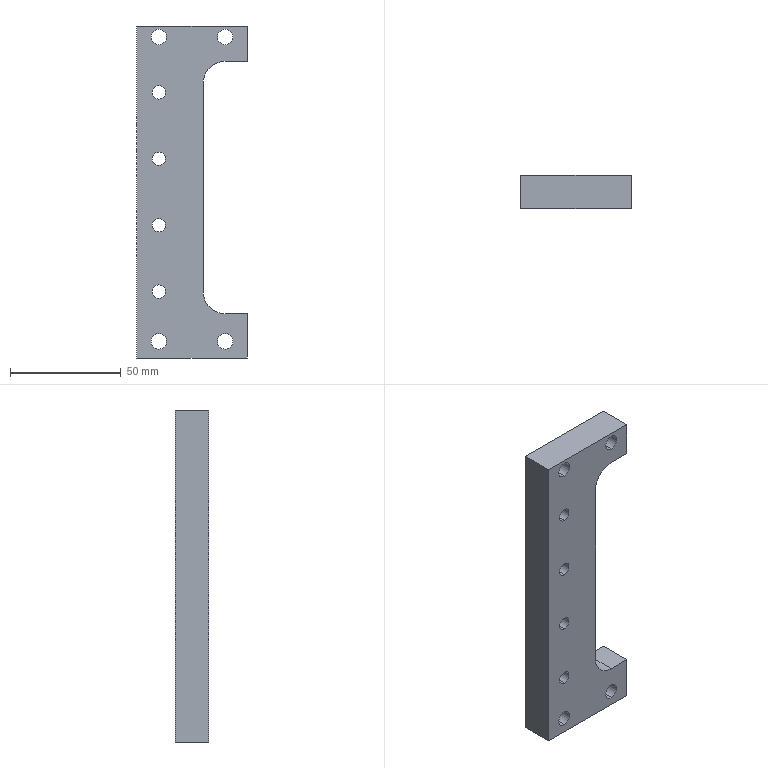Component | SolidWorks | JL001-05-05-001-1 | 1 solid | 28 faces | box 50 x 15 x 150 mm | volume 74938 mm3 | cylinder 18 | plane 10 | commonest cylinder face diameters 7 x8 6 x8 20 x2
build123d program:
from build123d import *

# Parameters (mm, degrees)
SKETCH1_W                    = 50
SKETCH1_H                    = 150
BOSS_EXTRUDE1_DEPTH          = 15
M6_TAPPED_HOLE1_D            = 6
F_7_0_7_DIAMETER_HOLE1_D     = 7
F_7_0_7_DIAMETER_HOLE1_DEPTH = 15
F_7_0_7_DIAMETER_HOLE1_TIP   = 2.103
SKETCH6_W                    = 20
SKETCH6_H                    = 114
CUT_EXTRUDE1_DEPTH           = 81.467
FILLET1_R                    = 10


with BuildPart() as part:
    # Sketch1 → Boss-Extrude1 (new body)
    with BuildSketch(Plane(origin=(0, 0, 0), x_dir=(1, 0, 0), z_dir=(0, 1, 0))):
        Rectangle(SKETCH1_W, SKETCH1_H)
    extrude(amount=BOSS_EXTRUDE1_DEPTH)

    # M6 Tapped Hole1 (through all)
    with Locations(Plane(origin=(0, 15, 0), x_dir=(1, 0, 0), z_dir=(0, 1, 0))):
        with Locations((-15, -15), (-15, -45), (-15, 15), (-15, 45)):
            Hole(M6_TAPPED_HOLE1_D / 2)

    # 7.0 _7_ Diameter Hole1
    with Locations(Plane(origin=(0, 15, 0), x_dir=(1, 0, 0), z_dir=(0, 1, 0))):
        with Locations((-15, -70), (15, -70), (-15, 67.5), (15, 67.5)):
            Hole(F_7_0_7_DIAMETER_HOLE1_D / 2, depth=F_7_0_7_DIAMETER_HOLE1_DEPTH)
            with Locations((0, 0, -(F_7_0_7_DIAMETER_HOLE1_DEPTH + F_7_0_7_DIAMETER_HOLE1_TIP / 2))):  # 118° drill point
                Cone(0, F_7_0_7_DIAMETER_HOLE1_D / 2, F_7_0_7_DIAMETER_HOLE1_TIP, mode=Mode.SUBTRACT)

    # Sketch6 → Cut-Extrude1 (cut, through all)
    with BuildSketch(Plane(origin=(0, 15, 0), x_dir=(1, 0, 0), z_dir=(0, 1, 0))):
        with Locations((15, -2)):
            Rectangle(SKETCH6_W, SKETCH6_H)
    extrude(amount=-CUT_EXTRUDE1_DEPTH, mode=Mode.SUBTRACT)

    # Fillet1
    fillet1_edges = [part.edges().sort_by_distance(p)[0] for p in [
        (5, 7.5, 59),
        (5, 7.5, -55),
    ]]
    fillet(fillet1_edges, radius=FILLET1_R)


solid = part.part

# Placed as in the assembly
solid = solid.moved(Location((0, -52.5, 67.5), (0, 0, 0)))
STEP:
#1=COLOUR_RGB('',0.7922,0.8196,0.9333);
#2=FILL_AREA_STYLE_COLOUR('',#1);
#3=FILL_AREA_STYLE('',(#2));
#4=SURFACE_STYLE_FILL_AREA(#3);
#5=SURFACE_SIDE_STYLE('',(#4));
#6=SURFACE_STYLE_USAGE(.BOTH.,#5);
#7=PRESENTATION_STYLE_ASSIGNMENT((#6));
#8=CARTESIAN_POINT('',(-0.5906,-2.067,5.276));
#9=VERTEX_POINT('',#8);
#10=CARTESIAN_POINT('',(-0.5906,-2.067,5.551));
#11=VERTEX_POINT('',#10);
#12=CARTESIAN_POINT('',(-0.5906,-2.067,5.413));
#13=DIRECTION('',(0.,1.,0.));
#14=DIRECTION('',(0.,0.,1.));
#15=AXIS2_PLACEMENT_3D('',#12,#13,#14);
#16=CIRCLE('',#15,0.1378);
#17=EDGE_CURVE('',#9,#11,#16,.T.);
#18=ORIENTED_EDGE('',*,*,#17,.F.);
#19=CARTESIAN_POINT('',(-0.5906,-1.476,5.276));
#20=VERTEX_POINT('',#19);
#21=CARTESIAN_POINT('',(-0.5906,-1.476,5.276));
#22=DIRECTION('',(0.,1.,0.));
#23=VECTOR('',#22,39.37);
#24=LINE('',#21,#23);
#25=EDGE_CURVE('',#9,#20,#24,.T.);
#26=ORIENTED_EDGE('',*,*,#25,.T.);
#27=CARTESIAN_POINT('',(-0.5906,-1.476,5.551));
#28=VERTEX_POINT('',#27);
#29=CARTESIAN_POINT('',(-0.5906,-1.476,5.413));
#30=DIRECTION('',(0.,1.,0.));
#31=DIRECTION('',(0.,0.,1.));
#32=AXIS2_PLACEMENT_3D('',#29,#30,#31);
#33=CIRCLE('',#32,0.1378);
#34=EDGE_CURVE('',#20,#28,#33,.T.);
#35=ORIENTED_EDGE('',*,*,#34,.T.);
#36=CARTESIAN_POINT('',(-0.5906,-1.476,5.551));
#37=DIRECTION('',(0.,1.,0.));
#38=VECTOR('',#37,39.37);
#39=LINE('',#36,#38);
#40=EDGE_CURVE('',#11,#28,#39,.T.);
#41=ORIENTED_EDGE('',*,*,#40,.F.);
#42=EDGE_LOOP('',(#18,#26,#35,#41));
#43=FACE_OUTER_BOUND('',#42,.T.);
#44=CARTESIAN_POINT('',(-0.5906,-1.476,5.413));
#45=DIRECTION('',(0.,1.,0.));
#46=DIRECTION('',(0.,0.,1.));
#47=AXIS2_PLACEMENT_3D('',#44,#45,#46);
#48=CYLINDRICAL_SURFACE('',#47,0.1378);
#49=ADVANCED_FACE('',(#43),#48,.F.);
#50=CARTESIAN_POINT('',(0.5906,-2.067,5.276));
#51=VERTEX_POINT('',#50);
#52=CARTESIAN_POINT('',(0.5906,-2.067,5.551));
#53=VERTEX_POINT('',#52);
#54=CARTESIAN_POINT('',(0.5906,-2.067,5.413));
#55=DIRECTION('',(0.,1.,0.));
#56=DIRECTION('',(0.,0.,1.));
#57=AXIS2_PLACEMENT_3D('',#54,#55,#56);
#58=CIRCLE('',#57,0.1378);
#59=EDGE_CURVE('',#51,#53,#58,.T.);
#60=ORIENTED_EDGE('',*,*,#59,.F.);
#61=CARTESIAN_POINT('',(0.5906,-1.476,5.276));
#62=VERTEX_POINT('',#61);
#63=CARTESIAN_POINT('',(0.5906,-1.476,5.276));
#64=DIRECTION('',(0.,1.,0.));
#65=VECTOR('',#64,39.37);
#66=LINE('',#63,#65);
#67=EDGE_CURVE('',#51,#62,#66,.T.);
#68=ORIENTED_EDGE('',*,*,#67,.T.);
#69=CARTESIAN_POINT('',(0.5906,-1.476,5.551));
#70=VERTEX_POINT('',#69);
#71=CARTESIAN_POINT('',(0.5906,-1.476,5.413));
#72=DIRECTION('',(0.,1.,0.));
#73=DIRECTION('',(0.,0.,1.));
#74=AXIS2_PLACEMENT_3D('',#71,#72,#73);
#75=CIRCLE('',#74,0.1378);
#76=EDGE_CURVE('',#62,#70,#75,.T.);
#77=ORIENTED_EDGE('',*,*,#76,.T.);
#78=CARTESIAN_POINT('',(0.5906,-1.476,5.551));
#79=DIRECTION('',(0.,1.,0.));
#80=VECTOR('',#79,39.37);
#81=LINE('',#78,#80);
#82=EDGE_CURVE('',#53,#70,#81,.T.);
#83=ORIENTED_EDGE('',*,*,#82,.F.);
#84=EDGE_LOOP('',(#60,#68,#77,#83));
#85=FACE_OUTER_BOUND('',#84,.T.);
#86=CARTESIAN_POINT('',(0.5906,-1.476,5.413));
#87=DIRECTION('',(0.,1.,0.));
#88=DIRECTION('',(0.,0.,1.));
#89=AXIS2_PLACEMENT_3D('',#86,#87,#88);
#90=CYLINDRICAL_SURFACE('',#89,0.1378);
#91=ADVANCED_FACE('',(#85),#90,.F.);
#92=CARTESIAN_POINT('',(-0.5906,-2.067,-0.1378));
#93=VERTEX_POINT('',#92);
#94=CARTESIAN_POINT('',(-0.5906,-2.067,0.1378));
#95=VERTEX_POINT('',#94);
#96=CARTESIAN_POINT('',(-0.5906,-2.067,0.));
#97=DIRECTION('',(0.,1.,0.));
#98=DIRECTION('',(0.,0.,1.));
#99=AXIS2_PLACEMENT_3D('',#96,#97,#98);
#100=CIRCLE('',#99,0.1378);
#101=EDGE_CURVE('',#93,#95,#100,.T.);
#102=ORIENTED_EDGE('',*,*,#101,.F.);
#103=CARTESIAN_POINT('',(-0.5906,-1.476,-0.1378));
#104=VERTEX_POINT('',#103);
#105=CARTESIAN_POINT('',(-0.5906,-1.476,-0.1378));
#106=DIRECTION('',(0.,1.,0.));
#107=VECTOR('',#106,39.37);
#108=LINE('',#105,#107);
#109=EDGE_CURVE('',#93,#104,#108,.T.);
#110=ORIENTED_EDGE('',*,*,#109,.T.);
#111=CARTESIAN_POINT('',(-0.5906,-1.476,0.1378));
#112=VERTEX_POINT('',#111);
#113=CARTESIAN_POINT('',(-0.5906,-1.476,0.));
#114=DIRECTION('',(0.,1.,0.));
#115=DIRECTION('',(0.,0.,1.));
#116=AXIS2_PLACEMENT_3D('',#113,#114,#115);
#117=CIRCLE('',#116,0.1378);
#118=EDGE_CURVE('',#104,#112,#117,.T.);
#119=ORIENTED_EDGE('',*,*,#118,.T.);
#120=CARTESIAN_POINT('',(-0.5906,-1.476,0.1378));
#121=DIRECTION('',(0.,1.,0.));
#122=VECTOR('',#121,39.37);
#123=LINE('',#120,#122);
#124=EDGE_CURVE('',#95,#112,#123,.T.);
#125=ORIENTED_EDGE('',*,*,#124,.F.);
#126=EDGE_LOOP('',(#102,#110,#119,#125));
#127=FACE_OUTER_BOUND('',#126,.T.);
#128=CARTESIAN_POINT('',(-0.5906,-1.476,0.));
#129=DIRECTION('',(0.,1.,0.));
#130=DIRECTION('',(0.,0.,1.));
#131=AXIS2_PLACEMENT_3D('',#128,#129,#130);
#132=CYLINDRICAL_SURFACE('',#131,0.1378);
#133=ADVANCED_FACE('',(#127),#132,.F.);
#134=CARTESIAN_POINT('',(0.5906,-2.067,-0.1378));
#135=VERTEX_POINT('',#134);
#136=CARTESIAN_POINT('',(0.5906,-2.067,0.1378));
#137=VERTEX_POINT('',#136);
#138=CARTESIAN_POINT('',(0.5906,-2.067,0.));
#139=DIRECTION('',(0.,1.,0.));
#140=DIRECTION('',(0.,0.,1.));
#141=AXIS2_PLACEMENT_3D('',#138,#139,#140);
#142=CIRCLE('',#141,0.1378);
#143=EDGE_CURVE('',#135,#137,#142,.T.);
#144=ORIENTED_EDGE('',*,*,#143,.F.);
#145=CARTESIAN_POINT('',(0.5906,-1.476,-0.1378));
#146=VERTEX_POINT('',#145);
#147=CARTESIAN_POINT('',(0.5906,-1.476,-0.1378));
#148=DIRECTION('',(0.,1.,0.));
#149=VECTOR('',#148,39.37);
#150=LINE('',#147,#149);
#151=EDGE_CURVE('',#135,#146,#150,.T.);
#152=ORIENTED_EDGE('',*,*,#151,.T.);
#153=CARTESIAN_POINT('',(0.5906,-1.476,0.1378));
#154=VERTEX_POINT('',#153);
#155=CARTESIAN_POINT('',(0.5906,-1.476,0.));
#156=DIRECTION('',(0.,1.,0.));
#157=DIRECTION('',(0.,0.,1.));
#158=AXIS2_PLACEMENT_3D('',#155,#156,#157);
#159=CIRCLE('',#158,0.1378);
#160=EDGE_CURVE('',#146,#154,#159,.T.);
#161=ORIENTED_EDGE('',*,*,#160,.T.);
#162=CARTESIAN_POINT('',(0.5906,-1.476,0.1378));
#163=DIRECTION('',(0.,1.,0.));
#164=VECTOR('',#163,39.37);
#165=LINE('',#162,#164);
#166=EDGE_CURVE('',#137,#154,#165,.T.);
#167=ORIENTED_EDGE('',*,*,#166,.F.);
#168=EDGE_LOOP('',(#144,#152,#161,#167));
#169=FACE_OUTER_BOUND('',#168,.T.);
#170=CARTESIAN_POINT('',(0.5906,-1.476,0.));
#171=DIRECTION('',(0.,1.,0.));
#172=DIRECTION('',(0.,0.,1.));
#173=AXIS2_PLACEMENT_3D('',#170,#171,#172);
#174=CYLINDRICAL_SURFACE('',#173,0.1378);
#175=ADVANCED_FACE('',(#169),#174,.F.);
#176=CARTESIAN_POINT('',(-0.5906,-2.067,3.13));
#177=VERTEX_POINT('',#176);
#178=CARTESIAN_POINT('',(-0.5906,-2.067,3.366));
#179=VERTEX_POINT('',#178);
#180=CARTESIAN_POINT('',(-0.5906,-2.067,3.248));
#181=DIRECTION('',(0.,1.,0.));
#182=DIRECTION('',(0.,0.,1.));
#183=AXIS2_PLACEMENT_3D('',#180,#181,#182);
#184=CIRCLE('',#183,0.1181);
#185=EDGE_CURVE('',#177,#179,#184,.T.);
#186=ORIENTED_EDGE('',*,*,#185,.F.);
#187=CARTESIAN_POINT('',(-0.5906,-1.476,3.13));
#188=VERTEX_POINT('',#187);
#189=CARTESIAN_POINT('',(-0.5906,-1.476,3.13));
#190=DIRECTION('',(0.,1.,0.));
#191=VECTOR('',#190,39.37);
#192=LINE('',#189,#191);
#193=EDGE_CURVE('',#177,#188,#192,.T.);
#194=ORIENTED_EDGE('',*,*,#193,.T.);
#195=CARTESIAN_POINT('',(-0.5906,-1.476,3.366));
#196=VERTEX_POINT('',#195);
#197=CARTESIAN_POINT('',(-0.5906,-1.476,3.248));
#198=DIRECTION('',(0.,1.,0.));
#199=DIRECTION('',(0.,0.,1.));
#200=AXIS2_PLACEMENT_3D('',#197,#198,#199);
#201=CIRCLE('',#200,0.1181);
#202=EDGE_CURVE('',#188,#196,#201,.T.);
#203=ORIENTED_EDGE('',*,*,#202,.T.);
#204=CARTESIAN_POINT('',(-0.5906,-1.476,3.366));
#205=DIRECTION('',(0.,1.,0.));
#206=VECTOR('',#205,39.37);
#207=LINE('',#204,#206);
#208=EDGE_CURVE('',#179,#196,#207,.T.);
#209=ORIENTED_EDGE('',*,*,#208,.F.);
#210=EDGE_LOOP('',(#186,#194,#203,#209));
#211=FACE_OUTER_BOUND('',#210,.T.);
#212=CARTESIAN_POINT('',(-0.5906,-1.476,3.248));
#213=DIRECTION('',(0.,1.,0.));
#214=DIRECTION('',(0.,0.,1.));
#215=AXIS2_PLACEMENT_3D('',#212,#213,#214);
#216=CYLINDRICAL_SURFACE('',#215,0.1181);
#217=ADVANCED_FACE('',(#211),#216,.F.);
#218=CARTESIAN_POINT('',(-0.5906,-2.067,4.311));
#219=VERTEX_POINT('',#218);
#220=CARTESIAN_POINT('',(-0.5906,-2.067,4.547));
#221=VERTEX_POINT('',#220);
#222=CARTESIAN_POINT('',(-0.5906,-2.067,4.429));
#223=DIRECTION('',(0.,1.,0.));
#224=DIRECTION('',(0.,0.,1.));
#225=AXIS2_PLACEMENT_3D('',#222,#223,#224);
#226=CIRCLE('',#225,0.1181);
#227=EDGE_CURVE('',#219,#221,#226,.T.);
#228=ORIENTED_EDGE('',*,*,#227,.F.);
#229=CARTESIAN_POINT('',(-0.5906,-1.476,4.311));
#230=VERTEX_POINT('',#229);
#231=CARTESIAN_POINT('',(-0.5906,-1.476,4.311));
#232=DIRECTION('',(0.,1.,0.));
#233=VECTOR('',#232,39.37);
#234=LINE('',#231,#233);
#235=EDGE_CURVE('',#219,#230,#234,.T.);
#236=ORIENTED_EDGE('',*,*,#235,.T.);
#237=CARTESIAN_POINT('',(-0.5906,-1.476,4.547));
#238=VERTEX_POINT('',#237);
#239=CARTESIAN_POINT('',(-0.5906,-1.476,4.429));
#240=DIRECTION('',(0.,1.,0.));
#241=DIRECTION('',(0.,0.,1.));
#242=AXIS2_PLACEMENT_3D('',#239,#240,#241);
#243=CIRCLE('',#242,0.1181);
#244=EDGE_CURVE('',#230,#238,#243,.T.);
#245=ORIENTED_EDGE('',*,*,#244,.T.);
#246=CARTESIAN_POINT('',(-0.5906,-1.476,4.547));
#247=DIRECTION('',(0.,1.,0.));
#248=VECTOR('',#247,39.37);
#249=LINE('',#246,#248);
#250=EDGE_CURVE('',#221,#238,#249,.T.);
#251=ORIENTED_EDGE('',*,*,#250,.F.);
#252=EDGE_LOOP('',(#228,#236,#245,#251));
#253=FACE_OUTER_BOUND('',#252,.T.);
#254=CARTESIAN_POINT('',(-0.5906,-1.476,4.429));
#255=DIRECTION('',(0.,1.,0.));
#256=DIRECTION('',(0.,0.,1.));
#257=AXIS2_PLACEMENT_3D('',#254,#255,#256);
#258=CYLINDRICAL_SURFACE('',#257,0.1181);
#259=ADVANCED_FACE('',(#253),#258,.F.);
#260=CARTESIAN_POINT('',(-0.5906,-2.067,1.949));
#261=VERTEX_POINT('',#260);
#262=CARTESIAN_POINT('',(-0.5906,-2.067,2.185));
#263=VERTEX_POINT('',#262);
#264=CARTESIAN_POINT('',(-0.5906,-2.067,2.067));
#265=DIRECTION('',(0.,1.,0.));
#266=DIRECTION('',(0.,0.,1.));
#267=AXIS2_PLACEMENT_3D('',#264,#265,#266);
#268=CIRCLE('',#267,0.1181);
#269=EDGE_CURVE('',#261,#263,#268,.T.);
#270=ORIENTED_EDGE('',*,*,#269,.F.);
#271=CARTESIAN_POINT('',(-0.5906,-1.476,1.949));
#272=VERTEX_POINT('',#271);
#273=CARTESIAN_POINT('',(-0.5906,-1.476,1.949));
#274=DIRECTION('',(0.,1.,0.));
#275=VECTOR('',#274,39.37);
#276=LINE('',#273,#275);
#277=EDGE_CURVE('',#261,#272,#276,.T.);
#278=ORIENTED_EDGE('',*,*,#277,.T.);
#279=CARTESIAN_POINT('',(-0.5906,-1.476,2.185));
#280=VERTEX_POINT('',#279);
#281=CARTESIAN_POINT('',(-0.5906,-1.476,2.067));
#282=DIRECTION('',(0.,1.,0.));
#283=DIRECTION('',(0.,0.,1.));
#284=AXIS2_PLACEMENT_3D('',#281,#282,#283);
#285=CIRCLE('',#284,0.1181);
#286=EDGE_CURVE('',#272,#280,#285,.T.);
#287=ORIENTED_EDGE('',*,*,#286,.T.);
#288=CARTESIAN_POINT('',(-0.5906,-1.476,2.185));
#289=DIRECTION('',(0.,1.,0.));
#290=VECTOR('',#289,39.37);
#291=LINE('',#288,#290);
#292=EDGE_CURVE('',#263,#280,#291,.T.);
#293=ORIENTED_EDGE('',*,*,#292,.F.);
#294=EDGE_LOOP('',(#270,#278,#287,#293));
#295=FACE_OUTER_BOUND('',#294,.T.);
#296=CARTESIAN_POINT('',(-0.5906,-1.476,2.067));
#297=DIRECTION('',(0.,1.,0.));
#298=DIRECTION('',(0.,0.,1.));
#299=AXIS2_PLACEMENT_3D('',#296,#297,#298);
#300=CYLINDRICAL_SURFACE('',#299,0.1181);
#301=ADVANCED_FACE('',(#295),#300,.F.);
#302=CARTESIAN_POINT('',(-0.5906,-2.067,0.7677));
#303=VERTEX_POINT('',#302);
#304=CARTESIAN_POINT('',(-0.5906,-2.067,1.004));
#305=VERTEX_POINT('',#304);
#306=CARTESIAN_POINT('',(-0.5906,-2.067,0.8858));
#307=DIRECTION('',(0.,1.,0.));
#308=DIRECTION('',(0.,0.,1.));
#309=AXIS2_PLACEMENT_3D('',#306,#307,#308);
#310=CIRCLE('',#309,0.1181);
#311=EDGE_CURVE('',#303,#305,#310,.T.);
#312=ORIENTED_EDGE('',*,*,#311,.F.);
#313=CARTESIAN_POINT('',(-0.5906,-1.476,0.7677));
#314=VERTEX_POINT('',#313);
#315=CARTESIAN_POINT('',(-0.5906,-1.476,0.7677));
#316=DIRECTION('',(0.,1.,0.));
#317=VECTOR('',#316,39.37);
#318=LINE('',#315,#317);
#319=EDGE_CURVE('',#303,#314,#318,.T.);
#320=ORIENTED_EDGE('',*,*,#319,.T.);
#321=CARTESIAN_POINT('',(-0.5906,-1.476,1.004));
#322=VERTEX_POINT('',#321);
#323=CARTESIAN_POINT('',(-0.5906,-1.476,0.8858));
#324=DIRECTION('',(0.,1.,0.));
#325=DIRECTION('',(0.,0.,1.));
#326=AXIS2_PLACEMENT_3D('',#323,#324,#325);
#327=CIRCLE('',#326,0.1181);
#328=EDGE_CURVE('',#314,#322,#327,.T.);
#329=ORIENTED_EDGE('',*,*,#328,.T.);
#330=CARTESIAN_POINT('',(-0.5906,-1.476,1.004));
#331=DIRECTION('',(0.,1.,0.));
#332=VECTOR('',#331,39.37);
#333=LINE('',#330,#332);
#334=EDGE_CURVE('',#305,#322,#333,.T.);
#335=ORIENTED_EDGE('',*,*,#334,.F.);
#336=EDGE_LOOP('',(#312,#320,#329,#335));
#337=FACE_OUTER_BOUND('',#336,.T.);
#338=CARTESIAN_POINT('',(-0.5906,-1.476,0.8858));
#339=DIRECTION('',(0.,1.,0.));
#340=DIRECTION('',(0.,0.,1.));
#341=AXIS2_PLACEMENT_3D('',#338,#339,#340);
#342=CYLINDRICAL_SURFACE('',#341,0.1181);
#343=ADVANCED_FACE('',(#337),#342,.F.);
#344=CARTESIAN_POINT('',(0.9843,-2.067,5.61));
#345=VERTEX_POINT('',#344);
#346=CARTESIAN_POINT('',(0.9843,-2.067,4.98));
#347=VERTEX_POINT('',#346);
#348=CARTESIAN_POINT('',(0.9843,-2.067,-0.2953));
#349=DIRECTION('',(-0.,0.,-1.));
#350=VECTOR('',#349,39.37);
#351=LINE('',#348,#350);
#352=EDGE_CURVE('',#345,#347,#351,.T.);
#353=ORIENTED_EDGE('',*,*,#352,.T.);
#354=CARTESIAN_POINT('',(0.9843,-1.476,4.98));
#355=VERTEX_POINT('',#354);
#356=CARTESIAN_POINT('',(0.9843,-2.067,4.98));
#357=DIRECTION('',(0.,1.,0.));
#358=VECTOR('',#357,39.37);
#359=LINE('',#356,#358);
#360=EDGE_CURVE('',#347,#355,#359,.T.);
#361=ORIENTED_EDGE('',*,*,#360,.T.);
#362=CARTESIAN_POINT('',(0.9843,-1.476,5.61));
#363=VERTEX_POINT('',#362);
#364=CARTESIAN_POINT('',(0.9843,-1.476,-0.2953));
#365=DIRECTION('',(-0.,0.,-1.));
#366=VECTOR('',#365,39.37);
#367=LINE('',#364,#366);
#368=EDGE_CURVE('',#363,#355,#367,.T.);
#369=ORIENTED_EDGE('',*,*,#368,.F.);
#370=CARTESIAN_POINT('',(0.9843,-1.476,5.61));
#371=DIRECTION('',(0.,-1.,0.));
#372=VECTOR('',#371,39.37);
#373=LINE('',#370,#372);
#374=EDGE_CURVE('',#363,#345,#373,.T.);
#375=ORIENTED_EDGE('',*,*,#374,.T.);
#376=EDGE_LOOP('',(#353,#361,#369,#375));
#377=FACE_OUTER_BOUND('',#376,.T.);
#378=CARTESIAN_POINT('',(0.9843,-1.476,-0.2953));
#379=DIRECTION('',(-1.,0.,0.));
#380=DIRECTION('',(0.,0.,1.));
#381=AXIS2_PLACEMENT_3D('',#378,#379,#380);
#382=PLANE('',#381);
#383=ADVANCED_FACE('',(#377),#382,.F.);
#384=CARTESIAN_POINT('',(0.9843,-1.476,0.4921));
#385=VERTEX_POINT('',#384);
#386=CARTESIAN_POINT('',(0.9843,-1.476,-0.2953));
#387=VERTEX_POINT('',#386);
#388=CARTESIAN_POINT('',(0.9843,-1.476,-0.2953));
#389=DIRECTION('',(-0.,0.,-1.));
#390=VECTOR('',#389,39.37);
#391=LINE('',#388,#390);
#392=EDGE_CURVE('',#385,#387,#391,.T.);
#393=ORIENTED_EDGE('',*,*,#392,.F.);
#394=CARTESIAN_POINT('',(0.9843,-2.067,0.4921));
#395=VERTEX_POINT('',#394);
#396=CARTESIAN_POINT('',(0.9843,-2.067,0.4921));
#397=DIRECTION('',(0.,1.,0.));
#398=VECTOR('',#397,39.37);
#399=LINE('',#396,#398);
#400=EDGE_CURVE('',#395,#385,#399,.T.);
#401=ORIENTED_EDGE('',*,*,#400,.F.);
#402=CARTESIAN_POINT('',(0.9843,-2.067,-0.2953));
#403=VERTEX_POINT('',#402);
#404=CARTESIAN_POINT('',(0.9843,-2.067,-0.2953));
#405=DIRECTION('',(-0.,0.,-1.));
#406=VECTOR('',#405,39.37);
#407=LINE('',#404,#406);
#408=EDGE_CURVE('',#395,#403,#407,.T.);
#409=ORIENTED_EDGE('',*,*,#408,.T.);
#410=CARTESIAN_POINT('',(0.9843,-1.476,-0.2953));
#411=DIRECTION('',(0.,-1.,0.));
#412=VECTOR('',#411,39.37);
#413=LINE('',#410,#412);
#414=EDGE_CURVE('',#387,#403,#413,.T.);
#415=ORIENTED_EDGE('',*,*,#414,.F.);
#416=EDGE_LOOP('',(#393,#401,#409,#415));
#417=FACE_OUTER_BOUND('',#416,.T.);
#418=CARTESIAN_POINT('',(0.9843,-1.476,-0.2953));
#419=DIRECTION('',(-1.,0.,0.));
#420=DIRECTION('',(0.,0.,1.));
#421=AXIS2_PLACEMENT_3D('',#418,#419,#420);
#422=PLANE('',#421);
#423=ADVANCED_FACE('',(#417),#422,.F.);
#424=CARTESIAN_POINT('',(-0.9843,-2.067,-0.2953));
#425=VERTEX_POINT('',#424);
#426=CARTESIAN_POINT('',(-0.9843,-2.067,-0.2953));
#427=DIRECTION('',(-1.,0.,0.));
#428=VECTOR('',#427,39.37);
#429=LINE('',#426,#428);
#430=EDGE_CURVE('',#403,#425,#429,.T.);
#431=ORIENTED_EDGE('',*,*,#430,.T.);
#432=CARTESIAN_POINT('',(-0.9843,-1.476,-0.2953));
#433=VERTEX_POINT('',#432);
#434=CARTESIAN_POINT('',(-0.9843,-1.476,-0.2953));
#435=DIRECTION('',(0.,-1.,0.));
#436=VECTOR('',#435,39.37);
#437=LINE('',#434,#436);
#438=EDGE_CURVE('',#433,#425,#437,.T.);
#439=ORIENTED_EDGE('',*,*,#438,.F.);
#440=CARTESIAN_POINT('',(-0.9843,-1.476,-0.2953));
#441=DIRECTION('',(-1.,0.,0.));
#442=VECTOR('',#441,39.37);
#443=LINE('',#440,#442);
#444=EDGE_CURVE('',#387,#433,#443,.T.);
#445=ORIENTED_EDGE('',*,*,#444,.F.);
#446=ORIENTED_EDGE('',*,*,#414,.T.);
#447=EDGE_LOOP('',(#431,#439,#445,#446));
#448=FACE_OUTER_BOUND('',#447,.T.);
#449=CARTESIAN_POINT('',(-0.9843,-1.476,-0.2953));
#450=DIRECTION('',(0.,0.,1.));
#451=DIRECTION('',(1.,0.,0.));
#452=AXIS2_PLACEMENT_3D('',#449,#450,#451);
#453=PLANE('',#452);
#454=ADVANCED_FACE('',(#448),#453,.F.);
#455=CARTESIAN_POINT('',(-0.9843,-2.067,5.61));
#456=VERTEX_POINT('',#455);
#457=CARTESIAN_POINT('',(-0.9843,-2.067,-0.2953));
#458=DIRECTION('',(0.,0.,1.));
#459=VECTOR('',#458,39.37);
#460=LINE('',#457,#459);
#461=EDGE_CURVE('',#425,#456,#460,.T.);
#462=ORIENTED_EDGE('',*,*,#461,.T.);
#463=CARTESIAN_POINT('',(-0.9843,-1.476,5.61));
#464=VERTEX_POINT('',#463);
#465=CARTESIAN_POINT('',(-0.9843,-1.476,5.61));
#466=DIRECTION('',(0.,-1.,0.));
#467=VECTOR('',#466,39.37);
#468=LINE('',#465,#467);
#469=EDGE_CURVE('',#464,#456,#468,.T.);
#470=ORIENTED_EDGE('',*,*,#469,.F.);
#471=CARTESIAN_POINT('',(-0.9843,-1.476,-0.2953));
#472=DIRECTION('',(0.,0.,1.));
#473=VECTOR('',#472,39.37);
#474=LINE('',#471,#473);
#475=EDGE_CURVE('',#433,#464,#474,.T.);
#476=ORIENTED_EDGE('',*,*,#475,.F.);
#477=ORIENTED_EDGE('',*,*,#438,.T.);
#478=EDGE_LOOP('',(#462,#470,#476,#477));
#479=FACE_OUTER_BOUND('',#478,.T.);
#480=CARTESIAN_POINT('',(-0.9843,-1.476,-0.2953));
#481=DIRECTION('',(1.,0.,-0.));
#482=DIRECTION('',(-0.,0.,-1.));
#483=AXIS2_PLACEMENT_3D('',#480,#481,#482);
#484=PLANE('',#483);
#485=ADVANCED_FACE('',(#479),#484,.F.);
#486=CARTESIAN_POINT('',(-0.9843,-2.067,5.61));
#487=DIRECTION('',(1.,0.,0.));
#488=VECTOR('',#487,39.37);
#489=LINE('',#486,#488);
#490=EDGE_CURVE('',#456,#345,#489,.T.);
#491=ORIENTED_EDGE('',*,*,#490,.T.);
#492=ORIENTED_EDGE('',*,*,#374,.F.);
#493=CARTESIAN_POINT('',(-0.9843,-1.476,5.61));
#494=DIRECTION('',(1.,0.,0.));
#495=VECTOR('',#494,39.37);
#496=LINE('',#493,#495);
#497=EDGE_CURVE('',#464,#363,#496,.T.);
#498=ORIENTED_EDGE('',*,*,#497,.F.);
#499=ORIENTED_EDGE('',*,*,#469,.T.);
#500=EDGE_LOOP('',(#491,#492,#498,#499));
#501=FACE_OUTER_BOUND('',#500,.T.);
#502=CARTESIAN_POINT('',(-0.9843,-1.476,5.61));
#503=DIRECTION('',(0.,0.,-1.));
#504=DIRECTION('',(-1.,0.,0.));
#505=AXIS2_PLACEMENT_3D('',#502,#503,#504);
#506=PLANE('',#505);
#507=ADVANCED_FACE('',(#501),#506,.F.);
#508=CARTESIAN_POINT('',(0.5906,-1.476,4.98));
#509=VERTEX_POINT('',#508);
#510=CARTESIAN_POINT('',(0.9843,-1.476,4.98));
#511=DIRECTION('',(1.,0.,0.));
#512=VECTOR('',#511,39.37);
#513=LINE('',#510,#512);
#514=EDGE_CURVE('',#509,#355,#513,.T.);
#515=ORIENTED_EDGE('',*,*,#514,.F.);
#516=CARTESIAN_POINT('',(0.1969,-1.476,4.587));
#517=VERTEX_POINT('',#516);
#518=CARTESIAN_POINT('',(0.5906,-1.476,4.587));
#519=DIRECTION('',(0.,-1.,0.));
#520=DIRECTION('',(0.,0.,1.));
#521=AXIS2_PLACEMENT_3D('',#518,#519,#520);
#522=CIRCLE('',#521,0.3937);
#523=EDGE_CURVE('',#509,#517,#522,.T.);
#524=ORIENTED_EDGE('',*,*,#523,.T.);
#525=CARTESIAN_POINT('',(0.1969,-1.476,0.8858));
#526=VERTEX_POINT('',#525);
#527=CARTESIAN_POINT('',(0.1969,-1.476,4.98));
#528=DIRECTION('',(0.,0.,1.));
#529=VECTOR('',#528,39.37);
#530=LINE('',#527,#529);
#531=EDGE_CURVE('',#526,#517,#530,.T.);
#532=ORIENTED_EDGE('',*,*,#531,.F.);
#533=CARTESIAN_POINT('',(0.5906,-1.476,0.4921));
#534=VERTEX_POINT('',#533);
#535=CARTESIAN_POINT('',(0.5906,-1.476,0.8858));
#536=DIRECTION('',(0.,-1.,0.));
#537=DIRECTION('',(0.,0.,1.));
#538=AXIS2_PLACEMENT_3D('',#535,#536,#537);
#539=CIRCLE('',#538,0.3937);
#540=EDGE_CURVE('',#526,#534,#539,.T.);
#541=ORIENTED_EDGE('',*,*,#540,.T.);
#542=CARTESIAN_POINT('',(0.9843,-1.476,0.4921));
#543=DIRECTION('',(-1.,0.,0.));
#544=VECTOR('',#543,39.37);
#545=LINE('',#542,#544);
#546=EDGE_CURVE('',#385,#534,#545,.T.);
#547=ORIENTED_EDGE('',*,*,#546,.F.);
#548=ORIENTED_EDGE('',*,*,#392,.T.);
#549=ORIENTED_EDGE('',*,*,#444,.T.);
#550=ORIENTED_EDGE('',*,*,#475,.T.);
#551=ORIENTED_EDGE('',*,*,#497,.T.);
#552=ORIENTED_EDGE('',*,*,#368,.T.);
#553=EDGE_LOOP('',(#515,#524,#532,#541,#547,#548,#549,#550,#551,#552));
#554=FACE_OUTER_BOUND('',#553,.T.);
#555=CARTESIAN_POINT('',(-0.5906,-1.476,5.413));
#556=DIRECTION('',(0.,1.,0.));
#557=DIRECTION('',(0.,0.,1.));
#558=AXIS2_PLACEMENT_3D('',#555,#556,#557);
#559=CIRCLE('',#558,0.1378);
#560=EDGE_CURVE('',#28,#20,#559,.T.);
#561=ORIENTED_EDGE('',*,*,#560,.F.);
#562=ORIENTED_EDGE('',*,*,#34,.F.);
#563=EDGE_LOOP('',(#561,#562));
#564=FACE_BOUND('',#563,.T.);
#565=CARTESIAN_POINT('',(0.5906,-1.476,5.413));
#566=DIRECTION('',(0.,1.,0.));
#567=DIRECTION('',(0.,0.,1.));
#568=AXIS2_PLACEMENT_3D('',#565,#566,#567);
#569=CIRCLE('',#568,0.1378);
#570=EDGE_CURVE('',#70,#62,#569,.T.);
#571=ORIENTED_EDGE('',*,*,#570,.F.);
#572=ORIENTED_EDGE('',*,*,#76,.F.);
#573=EDGE_LOOP('',(#571,#572));
#574=FACE_BOUND('',#573,.T.);
#575=CARTESIAN_POINT('',(-0.5906,-1.476,0.));
#576=DIRECTION('',(0.,1.,0.));
#577=DIRECTION('',(0.,0.,1.));
#578=AXIS2_PLACEMENT_3D('',#575,#576,#577);
#579=CIRCLE('',#578,0.1378);
#580=EDGE_CURVE('',#112,#104,#579,.T.);
#581=ORIENTED_EDGE('',*,*,#580,.F.);
#582=ORIENTED_EDGE('',*,*,#118,.F.);
#583=EDGE_LOOP('',(#581,#582));
#584=FACE_BOUND('',#583,.T.);
#585=CARTESIAN_POINT('',(0.5906,-1.476,0.));
#586=DIRECTION('',(0.,1.,0.));
#587=DIRECTION('',(0.,0.,1.));
#588=AXIS2_PLACEMENT_3D('',#585,#586,#587);
#589=CIRCLE('',#588,0.1378);
#590=EDGE_CURVE('',#154,#146,#589,.T.);
#591=ORIENTED_EDGE('',*,*,#590,.F.);
#592=ORIENTED_EDGE('',*,*,#160,.F.);
#593=EDGE_LOOP('',(#591,#592));
#594=FACE_BOUND('',#593,.T.);
#595=CARTESIAN_POINT('',(-0.5906,-1.476,3.248));
#596=DIRECTION('',(0.,1.,0.));
#597=DIRECTION('',(0.,0.,1.));
#598=AXIS2_PLACEMENT_3D('',#595,#596,#597);
#599=CIRCLE('',#598,0.1181);
#600=EDGE_CURVE('',#196,#188,#599,.T.);
#601=ORIENTED_EDGE('',*,*,#600,.F.);
#602=ORIENTED_EDGE('',*,*,#202,.F.);
#603=EDGE_LOOP('',(#601,#602));
#604=FACE_BOUND('',#603,.T.);
#605=CARTESIAN_POINT('',(-0.5906,-1.476,4.429));
#606=DIRECTION('',(0.,1.,0.));
#607=DIRECTION('',(0.,0.,1.));
#608=AXIS2_PLACEMENT_3D('',#605,#606,#607);
#609=CIRCLE('',#608,0.1181);
#610=EDGE_CURVE('',#238,#230,#609,.T.);
#611=ORIENTED_EDGE('',*,*,#610,.F.);
#612=ORIENTED_EDGE('',*,*,#244,.F.);
#613=EDGE_LOOP('',(#611,#612));
#614=FACE_BOUND('',#613,.T.);
#615=CARTESIAN_POINT('',(-0.5906,-1.476,2.067));
#616=DIRECTION('',(0.,1.,0.));
#617=DIRECTION('',(0.,0.,1.));
#618=AXIS2_PLACEMENT_3D('',#615,#616,#617);
#619=CIRCLE('',#618,0.1181);
#620=EDGE_CURVE('',#280,#272,#619,.T.);
#621=ORIENTED_EDGE('',*,*,#620,.F.);
#622=ORIENTED_EDGE('',*,*,#286,.F.);
#623=EDGE_LOOP('',(#621,#622));
#624=FACE_BOUND('',#623,.T.);
#625=CARTESIAN_POINT('',(-0.5906,-1.476,0.8858));
#626=DIRECTION('',(0.,1.,0.));
#627=DIRECTION('',(0.,0.,1.));
#628=AXIS2_PLACEMENT_3D('',#625,#626,#627);
#629=CIRCLE('',#628,0.1181);
#630=EDGE_CURVE('',#322,#314,#629,.T.);
#631=ORIENTED_EDGE('',*,*,#630,.F.);
#632=ORIENTED_EDGE('',*,*,#328,.F.);
#633=EDGE_LOOP('',(#631,#632));
#634=FACE_BOUND('',#633,.T.);
#635=CARTESIAN_POINT('',(0.,-1.476,2.657));
#636=DIRECTION('',(0.,1.,0.));
#637=DIRECTION('',(0.,0.,1.));
#638=AXIS2_PLACEMENT_3D('',#635,#636,#637);
#639=PLANE('',#638);
#640=ADVANCED_FACE('',(#554,#564,#574,#584,#594,#604,#614,#624,#634),#639,.T.);
#641=CARTESIAN_POINT('',(-0.5906,-2.067,5.413));
#642=DIRECTION('',(0.,1.,0.));
#643=DIRECTION('',(0.,0.,1.));
#644=AXIS2_PLACEMENT_3D('',#641,#642,#643);
#645=CIRCLE('',#644,0.1378);
#646=EDGE_CURVE('',#11,#9,#645,.T.);
#647=ORIENTED_EDGE('',*,*,#646,.T.);
#648=ORIENTED_EDGE('',*,*,#17,.T.);
#649=EDGE_LOOP('',(#647,#648));
#650=FACE_BOUND('',#649,.T.);
#651=CARTESIAN_POINT('',(0.5906,-2.067,5.413));
#652=DIRECTION('',(0.,1.,0.));
#653=DIRECTION('',(0.,0.,1.));
#654=AXIS2_PLACEMENT_3D('',#651,#652,#653);
#655=CIRCLE('',#654,0.1378);
#656=EDGE_CURVE('',#53,#51,#655,.T.);
#657=ORIENTED_EDGE('',*,*,#656,.T.);
#658=ORIENTED_EDGE('',*,*,#59,.T.);
#659=EDGE_LOOP('',(#657,#658));
#660=FACE_BOUND('',#659,.T.);
#661=CARTESIAN_POINT('',(-0.5906,-2.067,0.));
#662=DIRECTION('',(0.,1.,0.));
#663=DIRECTION('',(0.,0.,1.));
#664=AXIS2_PLACEMENT_3D('',#661,#662,#663);
#665=CIRCLE('',#664,0.1378);
#666=EDGE_CURVE('',#95,#93,#665,.T.);
#667=ORIENTED_EDGE('',*,*,#666,.T.);
#668=ORIENTED_EDGE('',*,*,#101,.T.);
#669=EDGE_LOOP('',(#667,#668));
#670=FACE_BOUND('',#669,.T.);
#671=CARTESIAN_POINT('',(0.5906,-2.067,0.));
#672=DIRECTION('',(0.,1.,0.));
#673=DIRECTION('',(0.,0.,1.));
#674=AXIS2_PLACEMENT_3D('',#671,#672,#673);
#675=CIRCLE('',#674,0.1378);
#676=EDGE_CURVE('',#137,#135,#675,.T.);
#677=ORIENTED_EDGE('',*,*,#676,.T.);
#678=ORIENTED_EDGE('',*,*,#143,.T.);
#679=EDGE_LOOP('',(#677,#678));
#680=FACE_BOUND('',#679,.T.);
#681=CARTESIAN_POINT('',(-0.5906,-2.067,3.248));
#682=DIRECTION('',(0.,1.,0.));
#683=DIRECTION('',(0.,0.,1.));
#684=AXIS2_PLACEMENT_3D('',#681,#682,#683);
#685=CIRCLE('',#684,0.1181);
#686=EDGE_CURVE('',#179,#177,#685,.T.);
#687=ORIENTED_EDGE('',*,*,#686,.T.);
#688=ORIENTED_EDGE('',*,*,#185,.T.);
#689=EDGE_LOOP('',(#687,#688));
#690=FACE_BOUND('',#689,.T.);
#691=CARTESIAN_POINT('',(-0.5906,-2.067,4.429));
#692=DIRECTION('',(0.,1.,0.));
#693=DIRECTION('',(0.,0.,1.));
#694=AXIS2_PLACEMENT_3D('',#691,#692,#693);
#695=CIRCLE('',#694,0.1181);
#696=EDGE_CURVE('',#221,#219,#695,.T.);
#697=ORIENTED_EDGE('',*,*,#696,.T.);
#698=ORIENTED_EDGE('',*,*,#227,.T.);
#699=EDGE_LOOP('',(#697,#698));
#700=FACE_BOUND('',#699,.T.);
#701=CARTESIAN_POINT('',(-0.5906,-2.067,2.067));
#702=DIRECTION('',(0.,1.,0.));
#703=DIRECTION('',(0.,0.,1.));
#704=AXIS2_PLACEMENT_3D('',#701,#702,#703);
#705=CIRCLE('',#704,0.1181);
#706=EDGE_CURVE('',#263,#261,#705,.T.);
#707=ORIENTED_EDGE('',*,*,#706,.T.);
#708=ORIENTED_EDGE('',*,*,#269,.T.);
#709=EDGE_LOOP('',(#707,#708));
#710=FACE_BOUND('',#709,.T.);
#711=CARTESIAN_POINT('',(-0.5906,-2.067,0.8858));
#712=DIRECTION('',(0.,1.,0.));
#713=DIRECTION('',(0.,0.,1.));
#714=AXIS2_PLACEMENT_3D('',#711,#712,#713);
#715=CIRCLE('',#714,0.1181);
#716=EDGE_CURVE('',#305,#303,#715,.T.);
#717=ORIENTED_EDGE('',*,*,#716,.T.);
#718=ORIENTED_EDGE('',*,*,#311,.T.);
#719=EDGE_LOOP('',(#717,#718));
#720=FACE_BOUND('',#719,.T.);
#721=CARTESIAN_POINT('',(0.5906,-2.067,0.4921));
#722=VERTEX_POINT('',#721);
#723=CARTESIAN_POINT('',(0.9843,-2.067,0.4921));
#724=DIRECTION('',(-1.,0.,0.));
#725=VECTOR('',#724,39.37);
#726=LINE('',#723,#725);
#727=EDGE_CURVE('',#395,#722,#726,.T.);
#728=ORIENTED_EDGE('',*,*,#727,.T.);
#729=CARTESIAN_POINT('',(0.1969,-2.067,0.8858));
#730=VERTEX_POINT('',#729);
#731=CARTESIAN_POINT('',(0.5906,-2.067,0.8858));
#732=DIRECTION('',(0.,1.,0.));
#733=DIRECTION('',(0.,0.,1.));
#734=AXIS2_PLACEMENT_3D('',#731,#732,#733);
#735=CIRCLE('',#734,0.3937);
#736=EDGE_CURVE('',#722,#730,#735,.T.);
#737=ORIENTED_EDGE('',*,*,#736,.T.);
#738=CARTESIAN_POINT('',(0.1969,-2.067,4.587));
#739=VERTEX_POINT('',#738);
#740=CARTESIAN_POINT('',(0.1969,-2.067,4.98));
#741=DIRECTION('',(0.,0.,1.));
#742=VECTOR('',#741,39.37);
#743=LINE('',#740,#742);
#744=EDGE_CURVE('',#730,#739,#743,.T.);
#745=ORIENTED_EDGE('',*,*,#744,.T.);
#746=CARTESIAN_POINT('',(0.5906,-2.067,4.98));
#747=VERTEX_POINT('',#746);
#748=CARTESIAN_POINT('',(0.5906,-2.067,4.587));
#749=DIRECTION('',(0.,1.,0.));
#750=DIRECTION('',(0.,0.,1.));
#751=AXIS2_PLACEMENT_3D('',#748,#749,#750);
#752=CIRCLE('',#751,0.3937);
#753=EDGE_CURVE('',#739,#747,#752,.T.);
#754=ORIENTED_EDGE('',*,*,#753,.T.);
#755=CARTESIAN_POINT('',(0.9843,-2.067,4.98));
#756=DIRECTION('',(1.,0.,0.));
#757=VECTOR('',#756,39.37);
#758=LINE('',#755,#757);
#759=EDGE_CURVE('',#747,#347,#758,.T.);
#760=ORIENTED_EDGE('',*,*,#759,.T.);
#761=ORIENTED_EDGE('',*,*,#352,.F.);
#762=ORIENTED_EDGE('',*,*,#490,.F.);
#763=ORIENTED_EDGE('',*,*,#461,.F.);
#764=ORIENTED_EDGE('',*,*,#430,.F.);
#765=ORIENTED_EDGE('',*,*,#408,.F.);
#766=EDGE_LOOP('',(#728,#737,#745,#754,#760,#761,#762,#763,#764,#765));
#767=FACE_OUTER_BOUND('',#766,.T.);
#768=CARTESIAN_POINT('',(0.,-2.067,2.657));
#769=DIRECTION('',(0.,1.,0.));
#770=DIRECTION('',(0.,0.,1.));
#771=AXIS2_PLACEMENT_3D('',#768,#769,#770);
#772=PLANE('',#771);
#773=ADVANCED_FACE('',(#650,#660,#670,#680,#690,#700,#710,#720,#767),#772,.F.);
#774=ORIENTED_EDGE('',*,*,#319,.F.);
#775=ORIENTED_EDGE('',*,*,#716,.F.);
#776=ORIENTED_EDGE('',*,*,#334,.T.);
#777=ORIENTED_EDGE('',*,*,#630,.T.);
#778=EDGE_LOOP('',(#774,#775,#776,#777));
#779=FACE_OUTER_BOUND('',#778,.T.);
#780=CARTESIAN_POINT('',(-0.5906,-1.476,0.8858));
#781=DIRECTION('',(0.,1.,0.));
#782=DIRECTION('',(0.,0.,1.));
#783=AXIS2_PLACEMENT_3D('',#780,#781,#782);
#784=CYLINDRICAL_SURFACE('',#783,0.1181);
#785=ADVANCED_FACE('',(#779),#784,.F.);
#786=ORIENTED_EDGE('',*,*,#277,.F.);
#787=ORIENTED_EDGE('',*,*,#706,.F.);
#788=ORIENTED_EDGE('',*,*,#292,.T.);
#789=ORIENTED_EDGE('',*,*,#620,.T.);
#790=EDGE_LOOP('',(#786,#787,#788,#789));
#791=FACE_OUTER_BOUND('',#790,.T.);
#792=CARTESIAN_POINT('',(-0.5906,-1.476,2.067));
#793=DIRECTION('',(0.,1.,0.));
#794=DIRECTION('',(0.,0.,1.));
#795=AXIS2_PLACEMENT_3D('',#792,#793,#794);
#796=CYLINDRICAL_SURFACE('',#795,0.1181);
#797=ADVANCED_FACE('',(#791),#796,.F.);
#798=ORIENTED_EDGE('',*,*,#235,.F.);
#799=ORIENTED_EDGE('',*,*,#696,.F.);
#800=ORIENTED_EDGE('',*,*,#250,.T.);
#801=ORIENTED_EDGE('',*,*,#610,.T.);
#802=EDGE_LOOP('',(#798,#799,#800,#801));
#803=FACE_OUTER_BOUND('',#802,.T.);
#804=CARTESIAN_POINT('',(-0.5906,-1.476,4.429));
#805=DIRECTION('',(0.,1.,0.));
#806=DIRECTION('',(0.,0.,1.));
#807=AXIS2_PLACEMENT_3D('',#804,#805,#806);
#808=CYLINDRICAL_SURFACE('',#807,0.1181);
#809=ADVANCED_FACE('',(#803),#808,.F.);
#810=ORIENTED_EDGE('',*,*,#193,.F.);
#811=ORIENTED_EDGE('',*,*,#686,.F.);
#812=ORIENTED_EDGE('',*,*,#208,.T.);
#813=ORIENTED_EDGE('',*,*,#600,.T.);
#814=EDGE_LOOP('',(#810,#811,#812,#813));
#815=FACE_OUTER_BOUND('',#814,.T.);
#816=CARTESIAN_POINT('',(-0.5906,-1.476,3.248));
#817=DIRECTION('',(0.,1.,0.));
#818=DIRECTION('',(0.,0.,1.));
#819=AXIS2_PLACEMENT_3D('',#816,#817,#818);
#820=CYLINDRICAL_SURFACE('',#819,0.1181);
#821=ADVANCED_FACE('',(#815),#820,.F.);
#822=ORIENTED_EDGE('',*,*,#151,.F.);
#823=ORIENTED_EDGE('',*,*,#676,.F.);
#824=ORIENTED_EDGE('',*,*,#166,.T.);
#825=ORIENTED_EDGE('',*,*,#590,.T.);
#826=EDGE_LOOP('',(#822,#823,#824,#825));
#827=FACE_OUTER_BOUND('',#826,.T.);
#828=CARTESIAN_POINT('',(0.5906,-1.476,0.));
#829=DIRECTION('',(0.,1.,0.));
#830=DIRECTION('',(0.,0.,1.));
#831=AXIS2_PLACEMENT_3D('',#828,#829,#830);
#832=CYLINDRICAL_SURFACE('',#831,0.1378);
#833=ADVANCED_FACE('',(#827),#832,.F.);
#834=ORIENTED_EDGE('',*,*,#109,.F.);
#835=ORIENTED_EDGE('',*,*,#666,.F.);
#836=ORIENTED_EDGE('',*,*,#124,.T.);
#837=ORIENTED_EDGE('',*,*,#580,.T.);
#838=EDGE_LOOP('',(#834,#835,#836,#837));
#839=FACE_OUTER_BOUND('',#838,.T.);
#840=CARTESIAN_POINT('',(-0.5906,-1.476,0.));
#841=DIRECTION('',(0.,1.,0.));
#842=DIRECTION('',(0.,0.,1.));
#843=AXIS2_PLACEMENT_3D('',#840,#841,#842);
#844=CYLINDRICAL_SURFACE('',#843,0.1378);
#845=ADVANCED_FACE('',(#839),#844,.F.);
#846=ORIENTED_EDGE('',*,*,#67,.F.);
#847=ORIENTED_EDGE('',*,*,#656,.F.);
#848=ORIENTED_EDGE('',*,*,#82,.T.);
#849=ORIENTED_EDGE('',*,*,#570,.T.);
#850=EDGE_LOOP('',(#846,#847,#848,#849));
#851=FACE_OUTER_BOUND('',#850,.T.);
#852=CARTESIAN_POINT('',(0.5906,-1.476,5.413));
#853=DIRECTION('',(0.,1.,0.));
#854=DIRECTION('',(0.,0.,1.));
#855=AXIS2_PLACEMENT_3D('',#852,#853,#854);
#856=CYLINDRICAL_SURFACE('',#855,0.1378);
#857=ADVANCED_FACE('',(#851),#856,.F.);
#858=ORIENTED_EDGE('',*,*,#25,.F.);
#859=ORIENTED_EDGE('',*,*,#646,.F.);
#860=ORIENTED_EDGE('',*,*,#40,.T.);
#861=ORIENTED_EDGE('',*,*,#560,.T.);
#862=EDGE_LOOP('',(#858,#859,#860,#861));
#863=FACE_OUTER_BOUND('',#862,.T.);
#864=CARTESIAN_POINT('',(-0.5906,-1.476,5.413));
#865=DIRECTION('',(0.,1.,0.));
#866=DIRECTION('',(0.,0.,1.));
#867=AXIS2_PLACEMENT_3D('',#864,#865,#866);
#868=CYLINDRICAL_SURFACE('',#867,0.1378);
#869=ADVANCED_FACE('',(#863),#868,.F.);
#870=ORIENTED_EDGE('',*,*,#759,.F.);
#871=CARTESIAN_POINT('',(0.5906,-1.476,4.98));
#872=DIRECTION('',(0.,1.,0.));
#873=VECTOR('',#872,39.37);
#874=LINE('',#871,#873);
#875=EDGE_CURVE('',#747,#509,#874,.T.);
#876=ORIENTED_EDGE('',*,*,#875,.T.);
#877=ORIENTED_EDGE('',*,*,#514,.T.);
#878=ORIENTED_EDGE('',*,*,#360,.F.);
#879=EDGE_LOOP('',(#870,#876,#877,#878));
#880=FACE_OUTER_BOUND('',#879,.T.);
#881=CARTESIAN_POINT('',(0.9843,-2.067,4.98));
#882=DIRECTION('',(0.,0.,1.));
#883=DIRECTION('',(1.,0.,0.));
#884=AXIS2_PLACEMENT_3D('',#881,#882,#883);
#885=PLANE('',#884);
#886=ADVANCED_FACE('',(#880),#885,.F.);
#887=ORIENTED_EDGE('',*,*,#531,.T.);
#888=CARTESIAN_POINT('',(0.1969,-2.067,4.587));
#889=DIRECTION('',(0.,-1.,0.));
#890=VECTOR('',#889,39.37);
#891=LINE('',#888,#890);
#892=EDGE_CURVE('',#517,#739,#891,.T.);
#893=ORIENTED_EDGE('',*,*,#892,.T.);
#894=ORIENTED_EDGE('',*,*,#744,.F.);
#895=CARTESIAN_POINT('',(0.1969,-1.476,0.8858));
#896=DIRECTION('',(0.,1.,0.));
#897=VECTOR('',#896,39.37);
#898=LINE('',#895,#897);
#899=EDGE_CURVE('',#730,#526,#898,.T.);
#900=ORIENTED_EDGE('',*,*,#899,.T.);
#901=EDGE_LOOP('',(#887,#893,#894,#900));
#902=FACE_OUTER_BOUND('',#901,.T.);
#903=CARTESIAN_POINT('',(0.1969,-2.067,4.98));
#904=DIRECTION('',(-1.,0.,0.));
#905=DIRECTION('',(0.,0.,1.));
#906=AXIS2_PLACEMENT_3D('',#903,#904,#905);
#907=PLANE('',#906);
#908=ADVANCED_FACE('',(#902),#907,.F.);
#909=ORIENTED_EDGE('',*,*,#546,.T.);
#910=CARTESIAN_POINT('',(0.5906,-2.067,0.4921));
#911=DIRECTION('',(0.,-1.,0.));
#912=VECTOR('',#911,39.37);
#913=LINE('',#910,#912);
#914=EDGE_CURVE('',#534,#722,#913,.T.);
#915=ORIENTED_EDGE('',*,*,#914,.T.);
#916=ORIENTED_EDGE('',*,*,#727,.F.);
#917=ORIENTED_EDGE('',*,*,#400,.T.);
#918=EDGE_LOOP('',(#909,#915,#916,#917));
#919=FACE_OUTER_BOUND('',#918,.T.);
#920=CARTESIAN_POINT('',(0.9843,-2.067,0.4921));
#921=DIRECTION('',(0.,0.,-1.));
#922=DIRECTION('',(-1.,0.,0.));
#923=AXIS2_PLACEMENT_3D('',#920,#921,#922);
#924=PLANE('',#923);
#925=ADVANCED_FACE('',(#919),#924,.F.);
#926=ORIENTED_EDGE('',*,*,#753,.F.);
#927=ORIENTED_EDGE('',*,*,#892,.F.);
#928=ORIENTED_EDGE('',*,*,#523,.F.);
#929=ORIENTED_EDGE('',*,*,#875,.F.);
#930=EDGE_LOOP('',(#926,#927,#928,#929));
#931=FACE_OUTER_BOUND('',#930,.T.);
#932=CARTESIAN_POINT('',(0.5906,-2.067,4.587));
#933=DIRECTION('',(0.,-1.,0.));
#934=DIRECTION('',(0.,0.,-1.));
#935=AXIS2_PLACEMENT_3D('',#932,#933,#934);
#936=CYLINDRICAL_SURFACE('',#935,0.3937);
#937=ADVANCED_FACE('',(#931),#936,.F.);
#938=ORIENTED_EDGE('',*,*,#736,.F.);
#939=ORIENTED_EDGE('',*,*,#914,.F.);
#940=ORIENTED_EDGE('',*,*,#540,.F.);
#941=ORIENTED_EDGE('',*,*,#899,.F.);
#942=EDGE_LOOP('',(#938,#939,#940,#941));
#943=FACE_OUTER_BOUND('',#942,.T.);
#944=CARTESIAN_POINT('',(0.5906,-2.067,0.8858));
#945=DIRECTION('',(0.,-1.,0.));
#946=DIRECTION('',(0.,0.,-1.));
#947=AXIS2_PLACEMENT_3D('',#944,#945,#946);
#948=CYLINDRICAL_SURFACE('',#947,0.3937);
#949=ADVANCED_FACE('',(#943),#948,.F.);
#950=CLOSED_SHELL('',(#49,#91,#133,#175,#217,#259,#301,#343,#383,#423,#454,#485,#507,#640,#773,#785,#797,#809,#821,#833,#845,#857,#869,#886,#908,#925,#937,#949));
#951=MANIFOLD_SOLID_BREP('',#950);
#952=STYLED_ITEM('',(#7),#951);
#953=PRESENTATION_LAYER_ASSIGNMENT('','',(#952));
#954=CARTESIAN_POINT('',(0.,0.,0.));
#955=DIRECTION('',(0.,0.,1.));
#956=DIRECTION('',(1.,0.,0.));
#957=AXIS2_PLACEMENT_3D('',#954,#955,#956);
#958=(LENGTH_UNIT()NAMED_UNIT(*)SI_UNIT($,.METRE.));
#959=LENGTH_MEASURE_WITH_UNIT(LENGTH_MEASURE(0.0254),#958);
#960=DIMENSIONAL_EXPONENTS(1.,0.,0.,0.,0.,0.,0.);
#961=(CONVERSION_BASED_UNIT('',#959)LENGTH_UNIT()NAMED_UNIT(#960));
#962=UNCERTAINTY_MEASURE_WITH_UNIT(LENGTH_MEASURE(0.00001),#961,'','');
#963=(NAMED_UNIT(*)PLANE_ANGLE_UNIT()SI_UNIT($,.RADIAN.));
#964=(NAMED_UNIT(*)SI_UNIT($,.STERADIAN.)SOLID_ANGLE_UNIT());
#965=(GEOMETRIC_REPRESENTATION_CONTEXT(3)GLOBAL_UNCERTAINTY_ASSIGNED_CONTEXT((#962))GLOBAL_UNIT_ASSIGNED_CONTEXT((#961,#963,#964))REPRESENTATION_CONTEXT('',''));
#966=ADVANCED_BREP_SHAPE_REPRESENTATION('',(#951,#957),#965);
#967=(LENGTH_UNIT()NAMED_UNIT(*)SI_UNIT($,.METRE.));
#968=LENGTH_MEASURE_WITH_UNIT(LENGTH_MEASURE(0.0254),#967);
#969=DIMENSIONAL_EXPONENTS(1.,0.,0.,0.,0.,0.,0.);
#970=(CONVERSION_BASED_UNIT('',#968)LENGTH_UNIT()NAMED_UNIT(#969));
#971=UNCERTAINTY_MEASURE_WITH_UNIT(LENGTH_MEASURE(0.00001),#970,'','');
#972=(NAMED_UNIT(*)PLANE_ANGLE_UNIT()SI_UNIT($,.RADIAN.));
#973=(NAMED_UNIT(*)SI_UNIT($,.STERADIAN.)SOLID_ANGLE_UNIT());
#974=(GEOMETRIC_REPRESENTATION_CONTEXT(3)GLOBAL_UNCERTAINTY_ASSIGNED_CONTEXT((#971))GLOBAL_UNIT_ASSIGNED_CONTEXT((#970,#972,#973))REPRESENTATION_CONTEXT('',''));
#975=MECHANICAL_DESIGN_GEOMETRIC_PRESENTATION_REPRESENTATION('',(#952),#974);